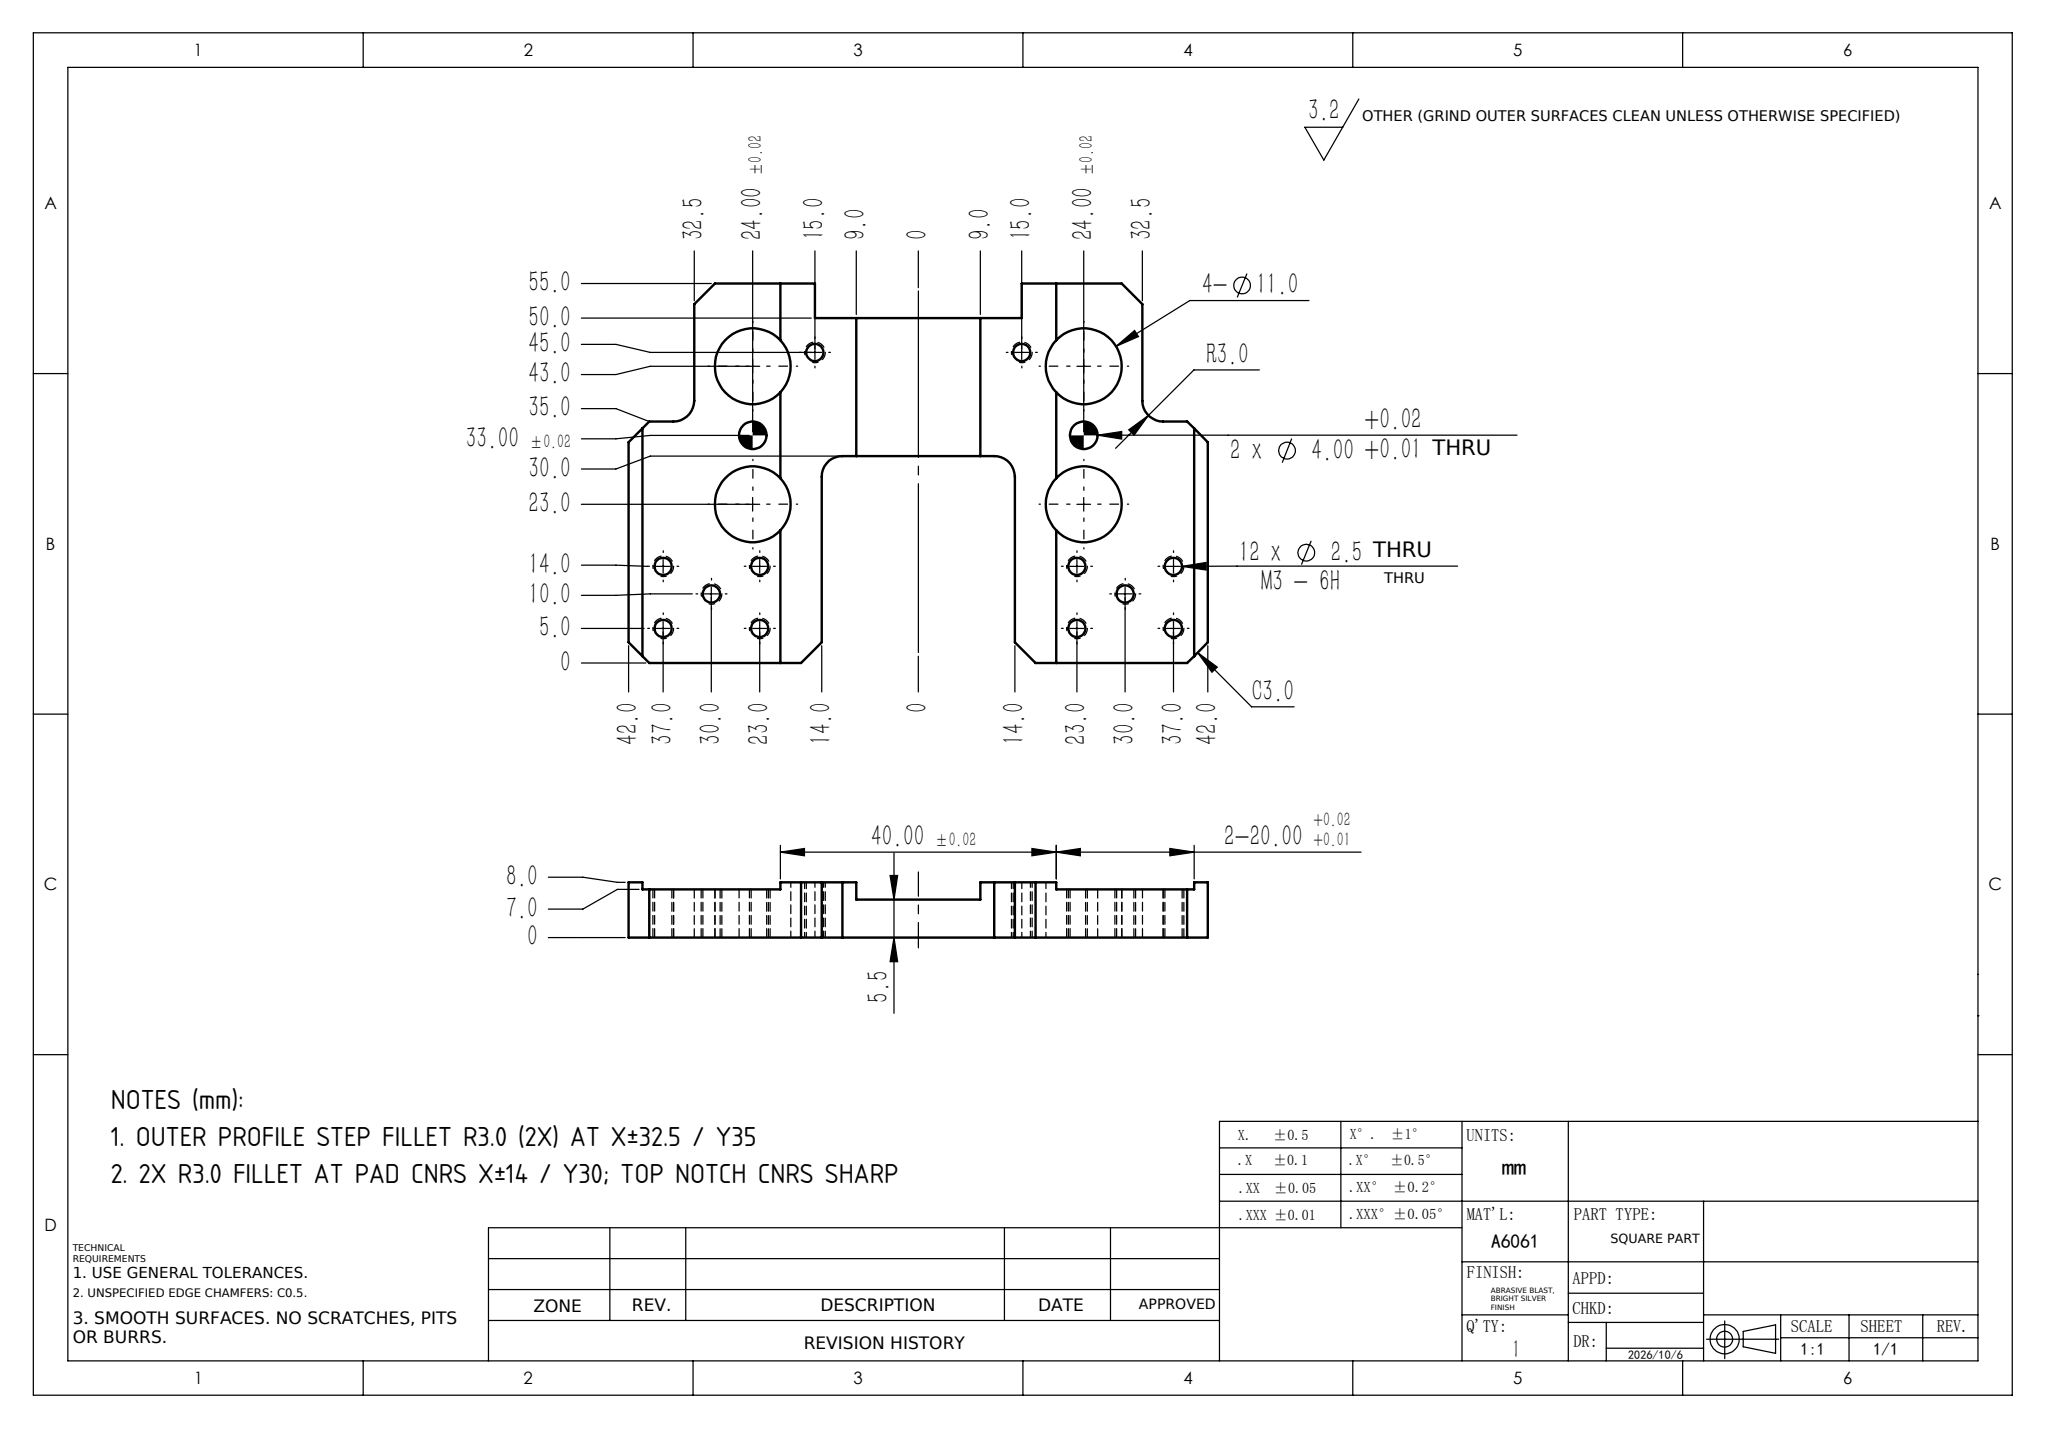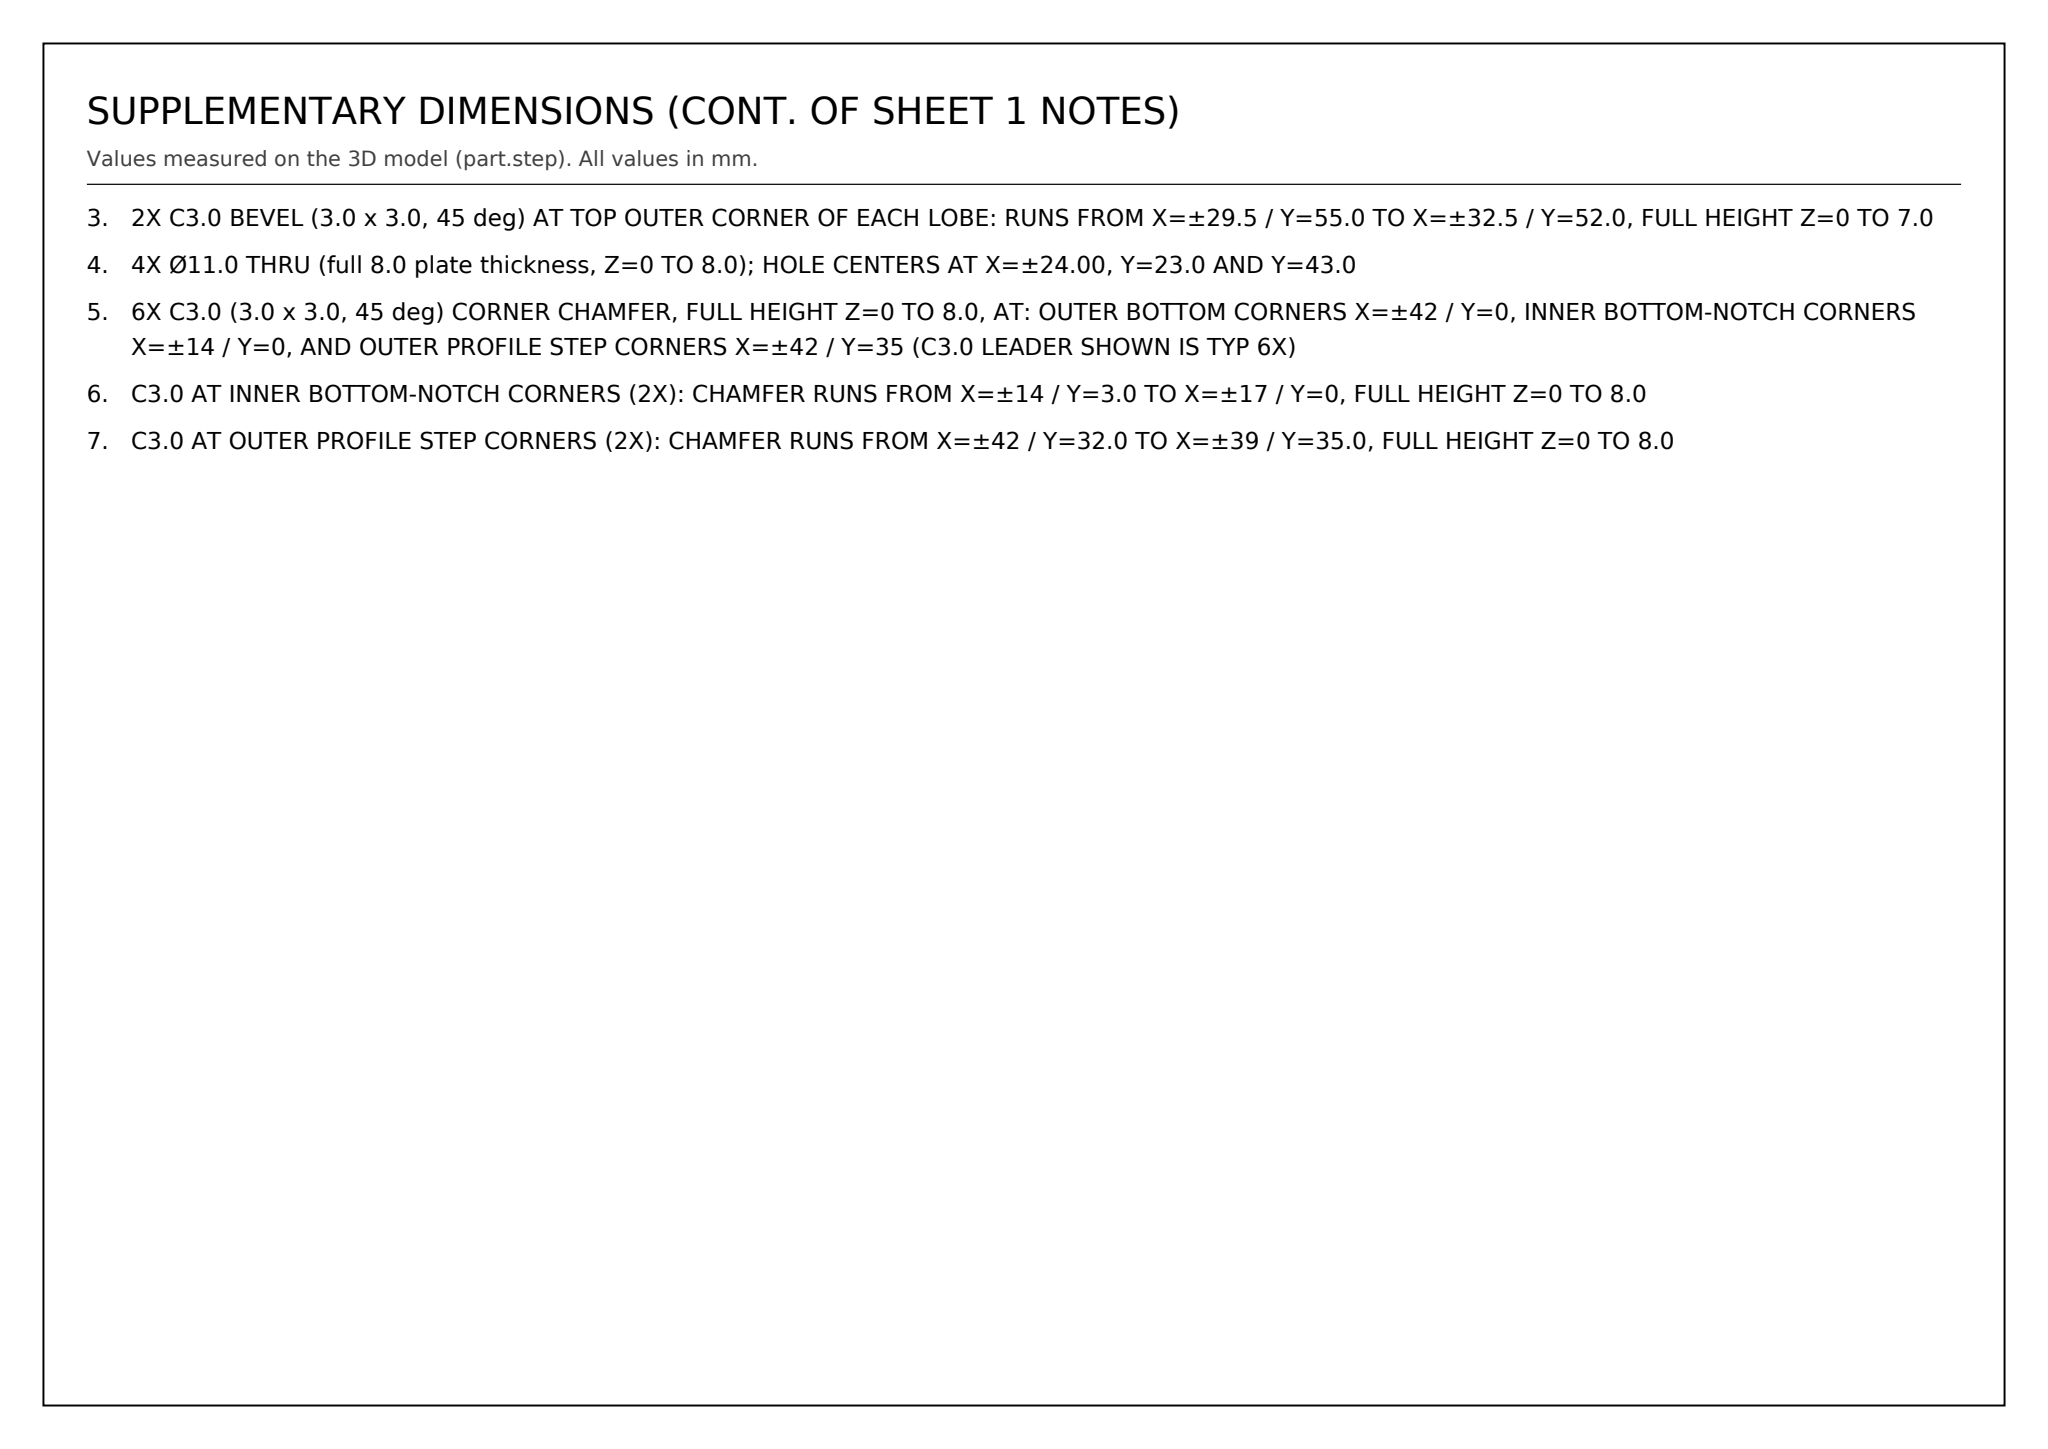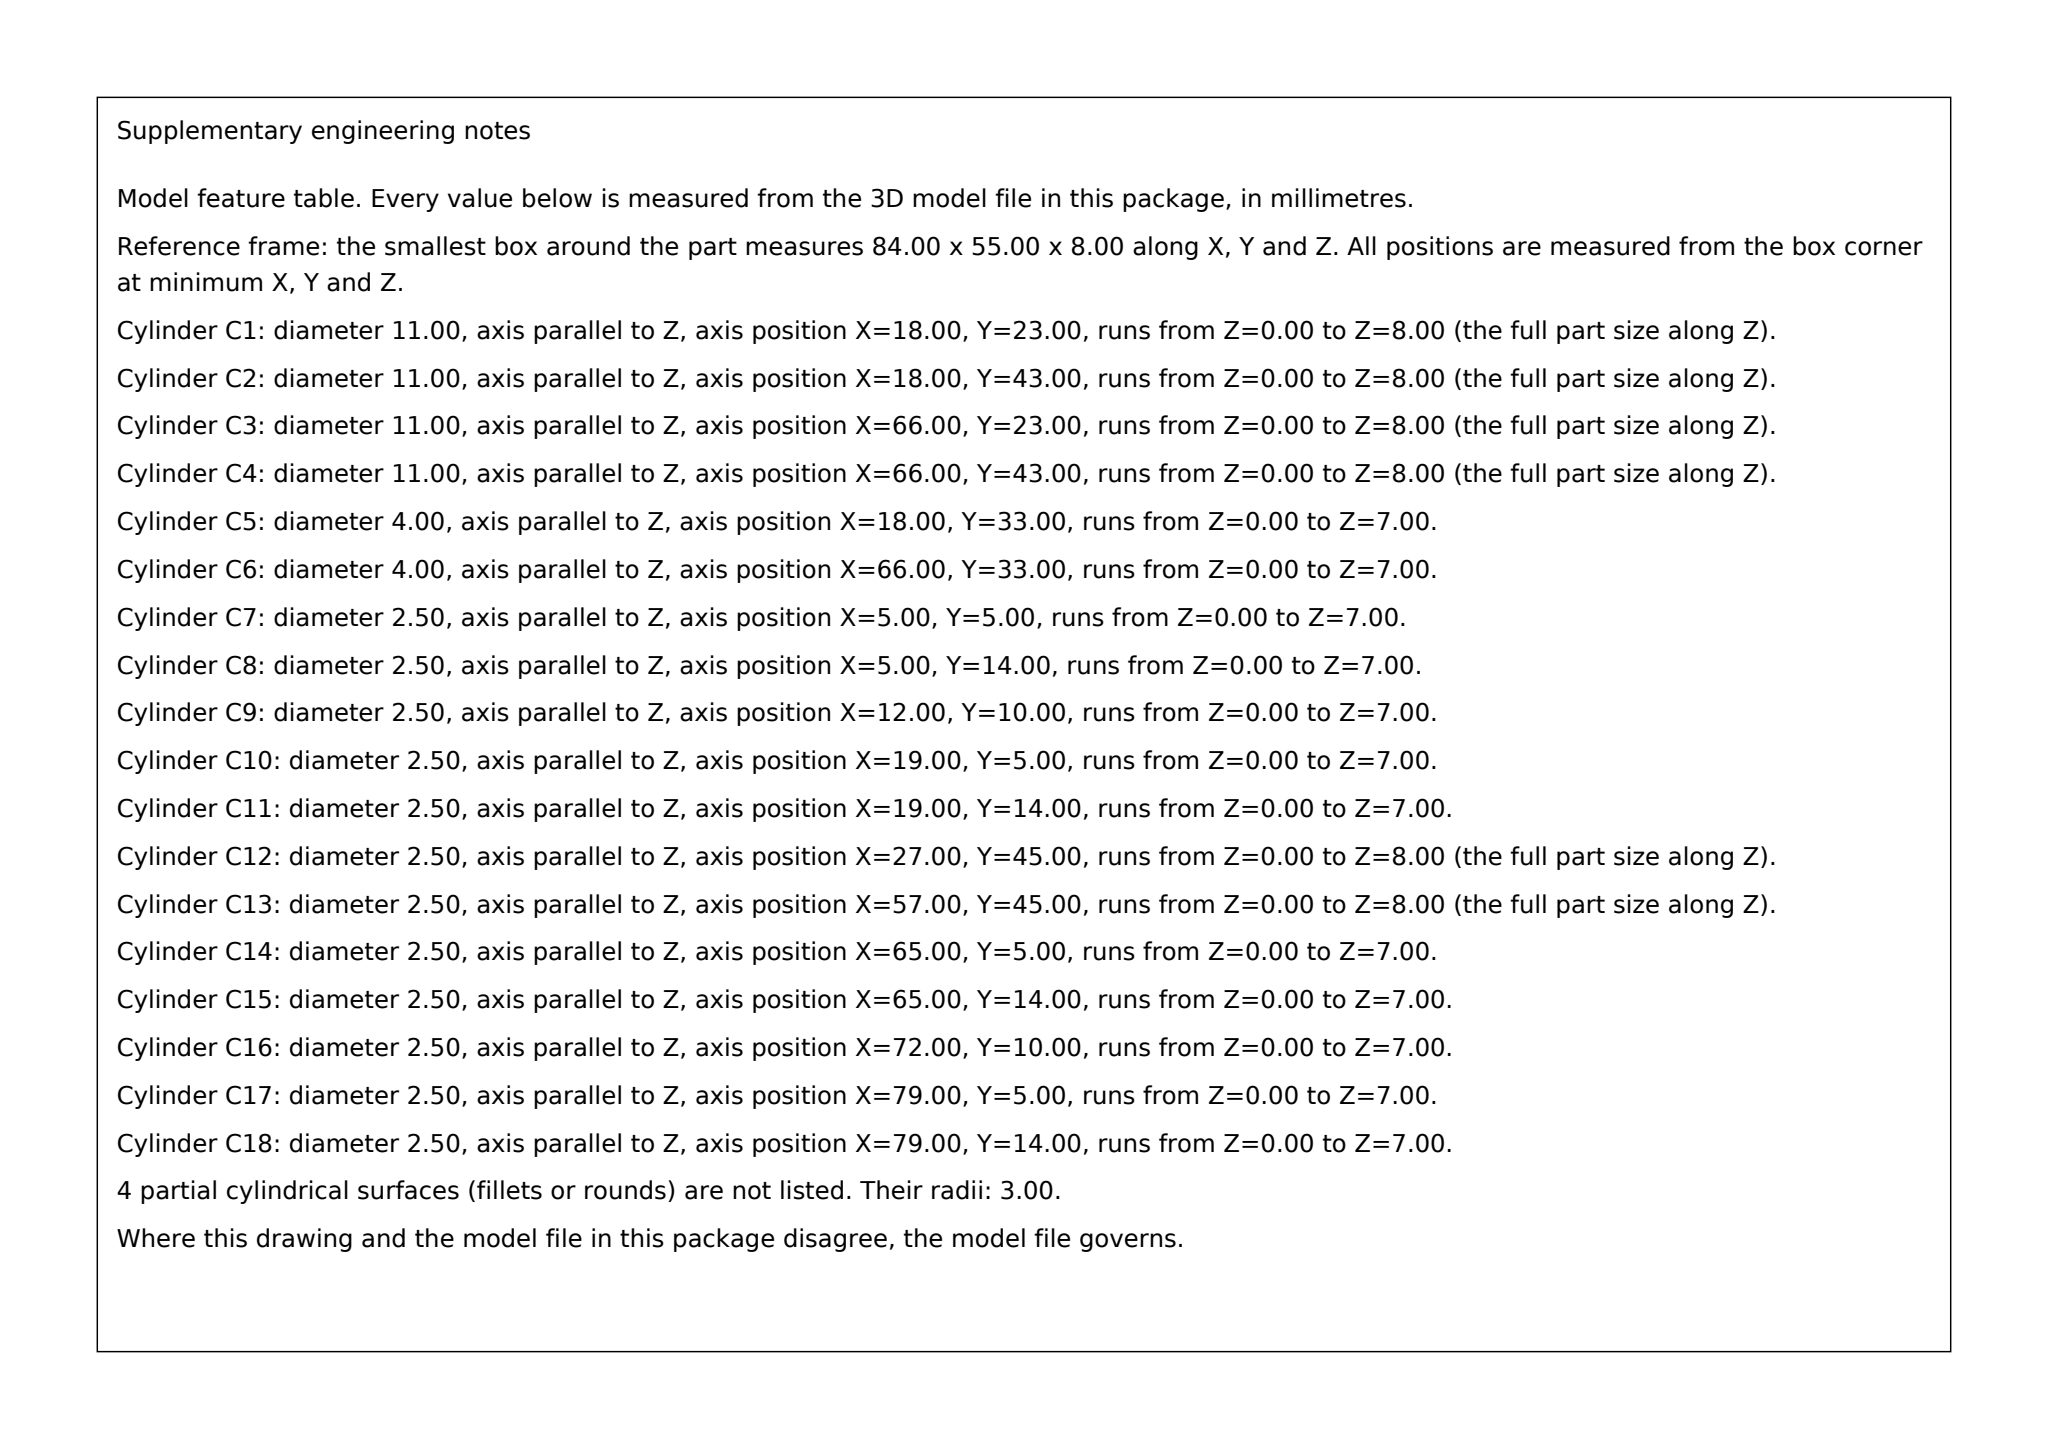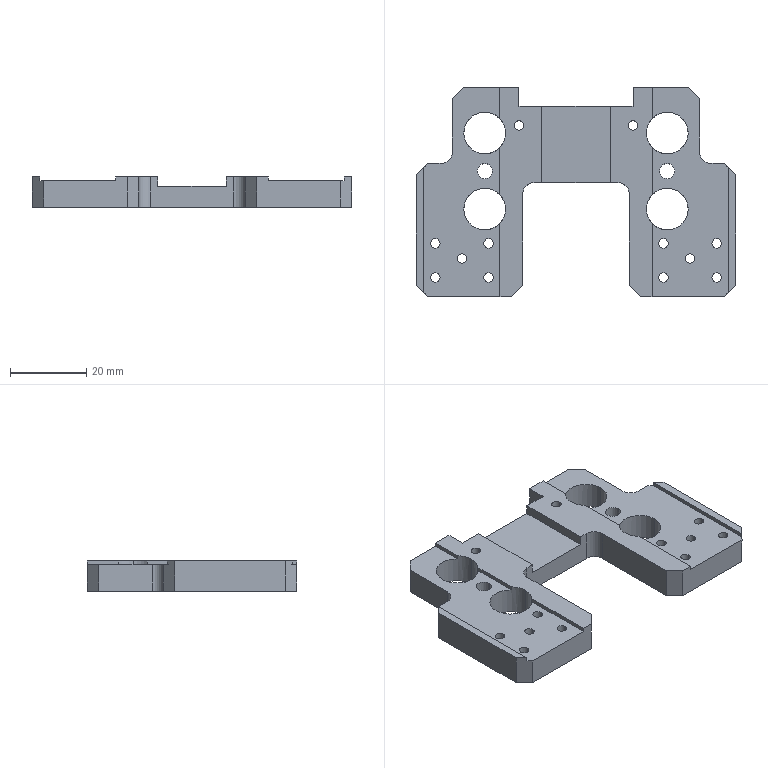Part | SolidWorks | mm | 1 solid | 82 faces | box 84 x 55 x 8 mm | volume 19691 mm3 | plane 42 | cylinder 40 | commonest cylinder face diameters 2.5 x24 11 x8 4 x4 6 x4
Drawing notes:
OUTER PROFILE STEP FILLET R3.0 (2X) AT X±32.5 / Y35 | from the solid: Dia 6.0 z-cylinders at (6.5,38) and (77.5,38), len 7.0, tangent to planes x=9.5/74.5 and y=35
2X R3.0 FILLET AT PAD CNRS X±14 / Y30; TOP NOTCH CNRS SHARP | from the solid: Dia 6.0 z-cylinders (R3.0) at (31,27) and (53,27), len 8.0, tangent to pad faces x=28/56 and y=30; no fillet cylinders at notch faces x=33/51, y=50
2X C3.0 BEVEL (3.0 x 3.0, 45 deg) AT TOP OUTER CORNER OF EACH LOBE: RUNS FROM X=±29.5 / Y=55.0 TO X=±32.5 / Y=52.0, FULL HEIGHT Z=0 TO 7.0 | from the solid: inclined_planes: angle_to_xyz_axes [45,45,90], bbox_from [9.5,52.0,0.0] and [71.5,52.0,0.0], size [3.0,3.0,7.0] (bbox 84.0 wide, X measured from center X=42.0; Y from bottom edge)
4X Ø11.0 THRU (full 8.0 plate thickness, Z=0 TO 8.0); HOLE CENTERS AT X=±24.00, Y=23.0 AND Y=43.0 | from the solid: cylinders: 4x hole/bore dia 11.0, axis z, at (18,23),(18,43),(66,23),(66,43), from 0.0 to 8.0; bbox_xyz z=8.0
6X C3.0 (3.0 x 3.0, 45 deg) CORNER CHAMFER, FULL HEIGHT Z=0 TO 8.0, AT: OUTER BOTTOM CORNERS X=±42 / Y=0, INNER BOTTOM-NOTCH CORNERS X=±14 / Y=0, AND OUTER PROFILE STEP CORNERS X=±42 / Y=35 (C3.0 LEADER SHOWN IS TYP 6X) | from the solid: inclined_planes: six 45/45/90 faces size 3.0x3.0x8.0 at bbox_from [0,0,0], [0,32,0], [25,0,0], [56,0,0], [81,0,0], [81,32,0] (bbox 84.0 x 55.0 x 8.0, X drawing = X step - 42)
C3.0 AT INNER BOTTOM-NOTCH CORNERS (2X): CHAMFER RUNS FROM X=±14 / Y=3.0 TO X=±17 / Y=0, FULL HEIGHT Z=0 TO 8.0 | from the solid: inclined_planes bbox_from [25,0,0] and [56,0,0], size [3.0,3.0,8.0] → X step 25-28 and 56-59, Y 0-3 (X drawing = X step - 42)
C3.0 AT OUTER PROFILE STEP CORNERS (2X): CHAMFER RUNS FROM X=±42 / Y=32.0 TO X=±39 / Y=35.0, FULL HEIGHT Z=0 TO 8.0 | from the solid: inclined_planes bbox_from [0,32,0] and [81,32,0], size [3.0,3.0,8.0] → X step 0-3 and 81-84, Y 32-35 (X drawing = X step - 42)
build123d program:
from build123d import *

# Parameters (mm, degrees)
SKETCH1_W                 = 84
SKETCH1_H                 = 55
BOSS_EXTRUDE1_DEPTH       = 8
SKETCH4_W                 = 28
SKETCH4_H                 = 30
SKETCH4_W_2               = 9.5
SKETCH4_H_2               = 20
CUT_EXTRUDE2_DEPTH        = 70.663
SKETCH2_W                 = 20
SKETCH2_H                 = 55
CUT_EXTRUDE1_DEPTH        = 1
SKETCH5_R                 = 5.5
CUT_EXTRUDE3_DEPTH        = 70.663
SIZE_MM_DOWEL_PIN_HOLE1_D = 4
M3_TAPPED_HOLE1_D         = 2.5
SKETCH15_W                = 30
SKETCH15_H                = 8
CUT_EXTRUDE5_DEPTH        = 5
SKETCH16_W                = 18
SKETCH16_H                = 20
CUT_EXTRUDE6_DEPTH        = 2.5
FILLET1_R                 = 3
CHAMFER1_SIZE             = 3


with BuildPart() as part:
    # Sketch1 → Boss-Extrude1 (new body)
    with BuildSketch(Plane.XY):
        with Locations((0, -27.5)):
            Rectangle(SKETCH1_W, SKETCH1_H)
    extrude(amount=BOSS_EXTRUDE1_DEPTH)

    # Sketch4 → Cut-Extrude2 (cut, through all)
    with BuildSketch(Plane.XY.offset(8)):
        with Locations((0, -40)):
            Rectangle(SKETCH4_W, SKETCH4_H)
        with Locations((37.25, -10)):
            Rectangle(SKETCH4_W_2, SKETCH4_H_2)
        with Locations((-37.25, -10)):
            Rectangle(SKETCH4_W_2, SKETCH4_H_2)
    extrude(amount=-CUT_EXTRUDE2_DEPTH, mode=Mode.SUBTRACT)

    # Sketch2 → Cut-Extrude1 (cut)
    with BuildSketch(Plane.XY.offset(8)):
        with Locations((-30, -27.5)):
            Rectangle(SKETCH2_W, SKETCH2_H)
        with Locations((30, -27.5)):
            Rectangle(SKETCH2_W, SKETCH2_H)
    extrude(amount=-CUT_EXTRUDE1_DEPTH, mode=Mode.SUBTRACT)

    # Sketch5 → Cut-Extrude3 (cut, through all)
    with BuildSketch(Plane.XY.offset(8)):
        with Locations((-24, -12)):
            Circle(SKETCH5_R)
        with Locations((24, -12)):
            Circle(SKETCH5_R)
        with Locations((-24, -32)):
            Circle(SKETCH5_R)
        with Locations((24, -32)):
            Circle(SKETCH5_R)
    extrude(amount=-CUT_EXTRUDE3_DEPTH, mode=Mode.SUBTRACT)

    # Size mm Dowel Pin Hole1 (through all)
    with Locations(Plane.XY.offset(7)):
        with Locations((-24, -22), (24, -22)):
            Hole(SIZE_MM_DOWEL_PIN_HOLE1_D / 2)

    # M3 Tapped Hole1 (through all)
    with Locations(Plane(origin=(0, 0, 0), x_dir=(-1, 0, 0), z_dir=(0, 0, -1))):
        with Locations((-15, -10), (15, -10), (30, -45), (-30, -45), (23, -41), (37, -41), (37, -50), (23, -50), (-37, -50), (-23, -50), (-23, -41), (-37, -41)):
            Hole(M3_TAPPED_HOLE1_D / 2)

    # Sketch15 → Cut-Extrude5 (cut)
    with BuildSketch(Plane(origin=(0, 0, 0), x_dir=(1, 0, 0), z_dir=(0, 1, 0))):
        with Locations((0, -4)):
            Rectangle(SKETCH15_W, SKETCH15_H)
    extrude(amount=-CUT_EXTRUDE5_DEPTH, mode=Mode.SUBTRACT)

    # Sketch16 → Cut-Extrude6 (cut)
    with BuildSketch(Plane.XY.offset(8)):
        with Locations((0, -15)):
            Rectangle(SKETCH16_W, SKETCH16_H)
    extrude(amount=-CUT_EXTRUDE6_DEPTH, mode=Mode.SUBTRACT)

    # Fillet1
    fillet1_edges = [part.edges().sort_by_distance(p)[0] for p in [
        (-14, -25, 4),
        (14, -25, 4),
        (32.5, -20, 3.5),
        (-32.5, -20, 3.5),
    ]]
    fillet(fillet1_edges, radius=FILLET1_R)

    # Chamfer1
    chamfer1_edges = [part.edges().sort_by_distance(p)[0] for p in [
        (42, -55, 4),
        (-42, -20, 4),
        (-42, -55, 4),
        (-14, -55, 4),
        (14, -55, 4),
        (32.5, 0, 3.5),
        (-32.5, 0, 3.5),
        (42, -20, 4),
    ]]
    chamfer(chamfer1_edges, length=CHAMFER1_SIZE)


solid = part.part